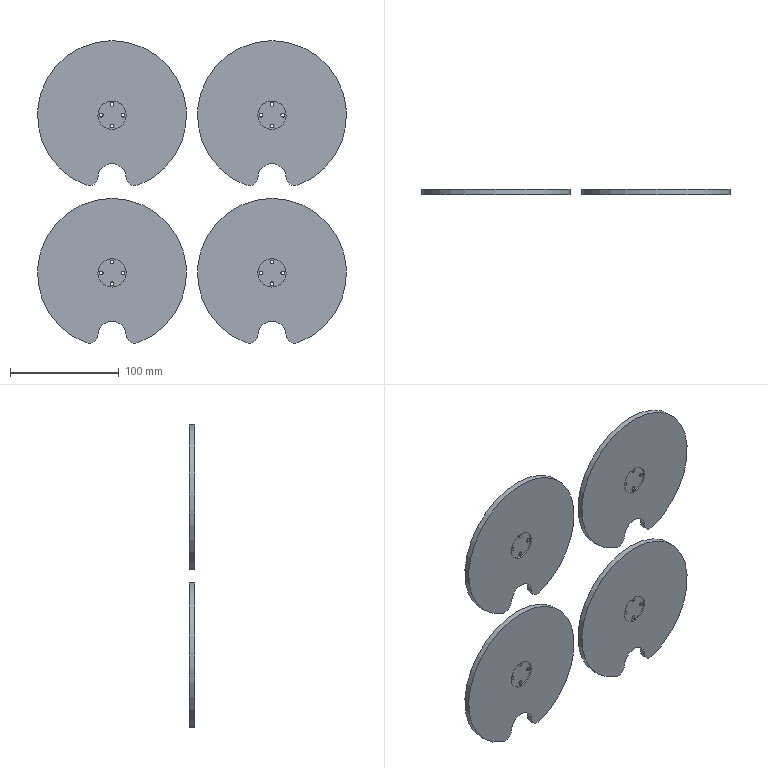CAM job | Mastercam | mm | 14 operations | part box 284 x 5 x 278.24
1. 2D High Speed (2D Area Mill) | 3 - 3 平铣刀
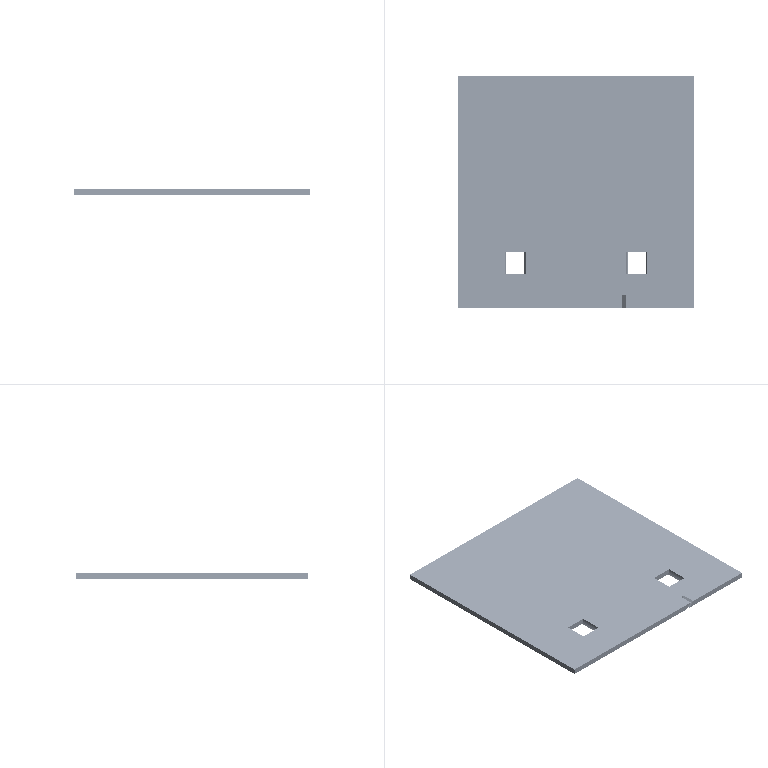2. 2D High Speed (2D Area Mill) | 3 - 3 平铣刀
3. Contour (2D) | 3 - 3 平铣刀
4. Contour (Ramp) | 3 - 3 平铣刀
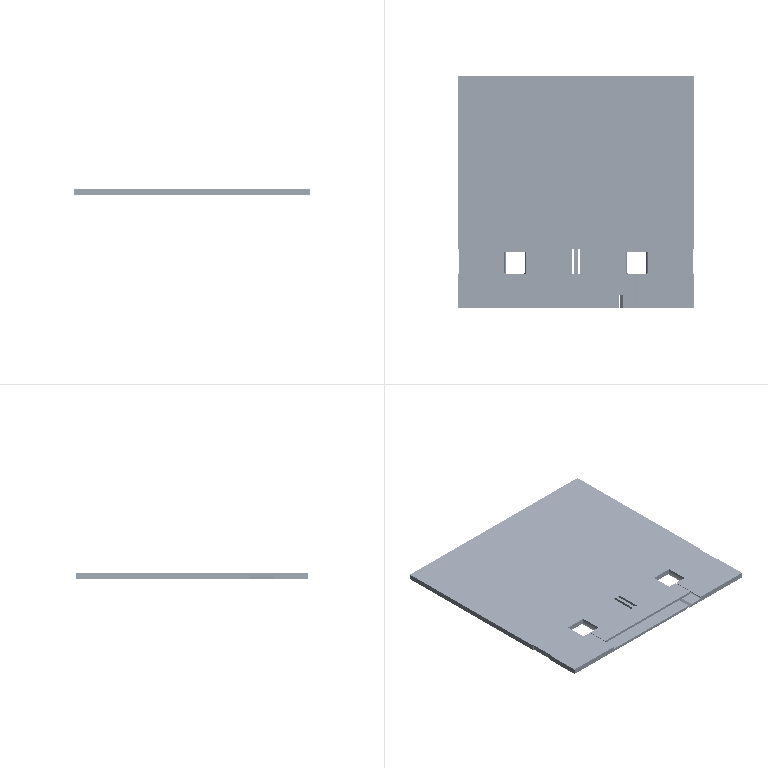5. Contour (2D) | 3 - 3 平铣刀
6. Drill/Counterbore | 7 - 4 倒角刀
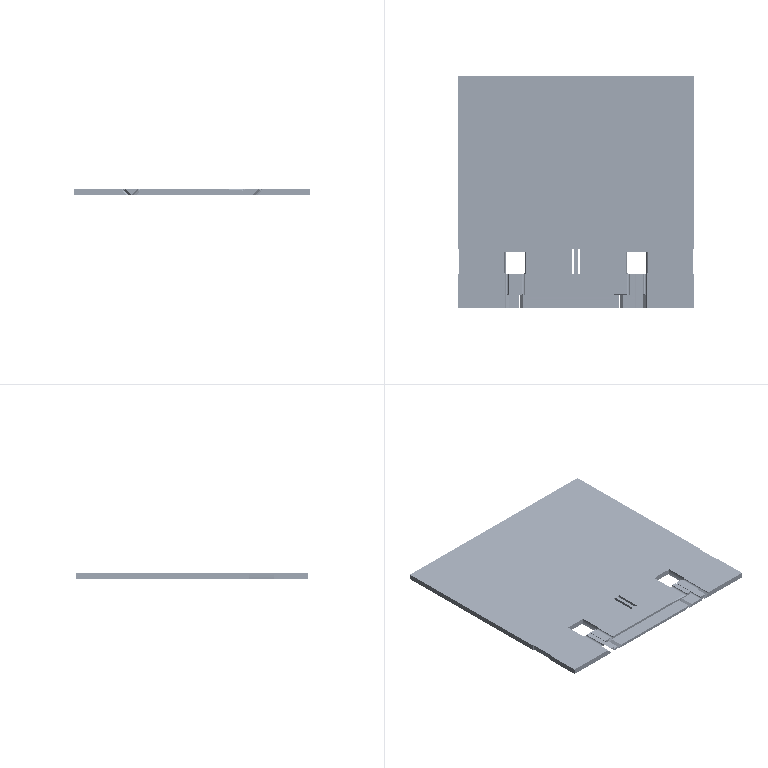7. Contour (2D chamfer) | 7 - 4 倒角刀
8. 2D High Speed (2D Area Mill) | 3 - 3 平铣刀
9. 2D High Speed (2D Area Mill) | 3 - 3 平铣刀
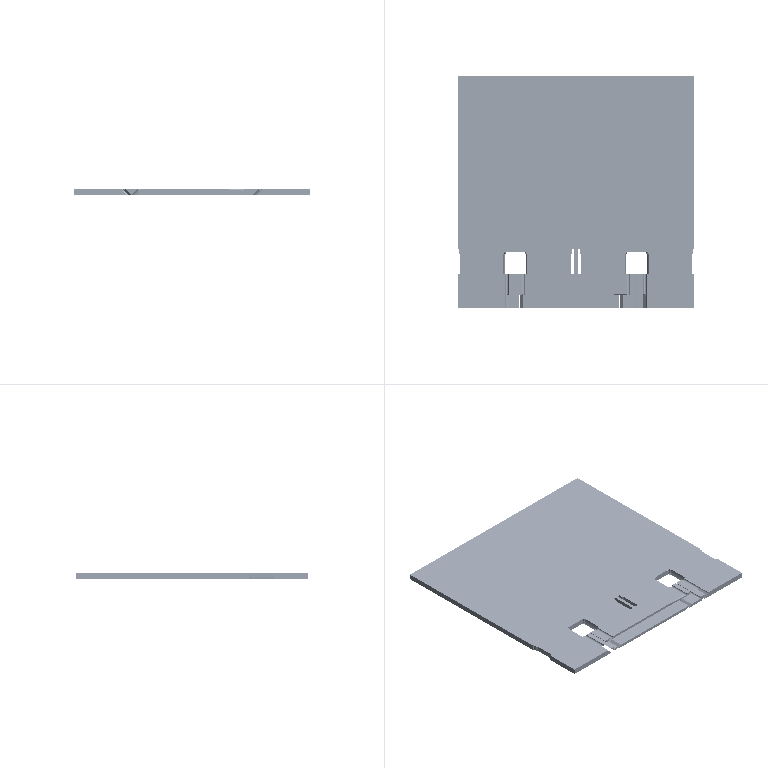10. Contour (2D) | 3 - 3 平铣刀
11. Contour (Ramp) | 3 - 3 平铣刀
12. Contour (2D) | 3 - 3 平铣刀
13. Drill/Counterbore | 7 - 4 倒角刀
14. Contour (2D chamfer) | 7 - 4 倒角刀